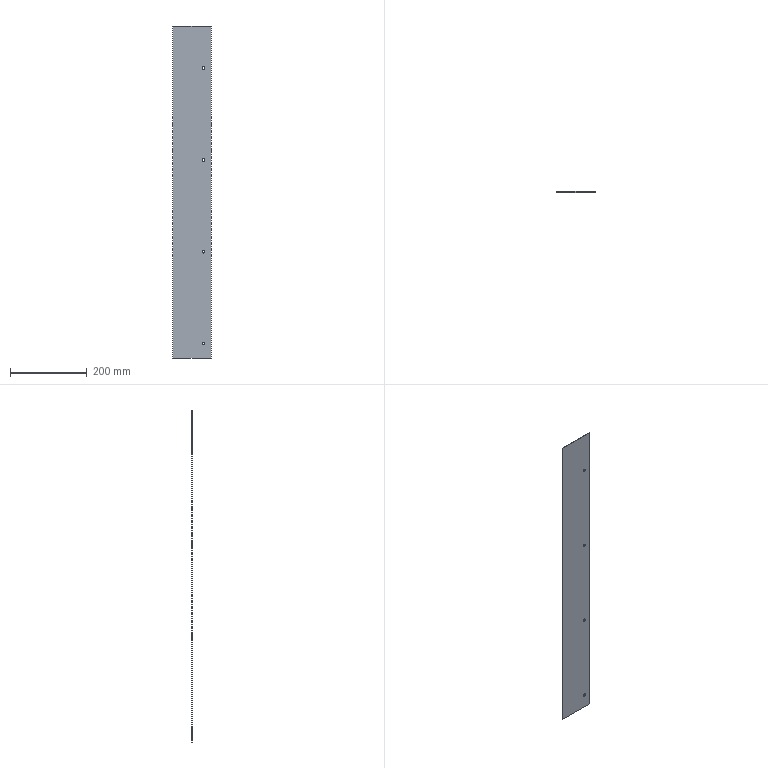Component | SolidWorks | 30-44A-1 | 1 solid | 14 faces | box 100 x 2 x 868 mm | volume 173292 mm3 | cylinder 8 | plane 6 | commonest cylinder face diameters 7 x8
STEP:
#1=COLOUR_RGB('',0.7922,0.8196,0.9333);
#2=FILL_AREA_STYLE_COLOUR('',#1);
#3=FILL_AREA_STYLE('',(#2));
#4=SURFACE_STYLE_FILL_AREA(#3);
#5=SURFACE_SIDE_STYLE('',(#4));
#6=SURFACE_STYLE_USAGE(.BOTH.,#5);
#7=PRESENTATION_STYLE_ASSIGNMENT((#6));
#8=CARTESIAN_POINT('',(10.731,28.038,-12.067));
#9=VERTEX_POINT('',#8);
#10=CARTESIAN_POINT('',(10.731,28.038,-12.343));
#11=VERTEX_POINT('',#10);
#12=CARTESIAN_POINT('',(10.731,28.038,-12.205));
#13=DIRECTION('',(-0.,-1.,0.));
#14=DIRECTION('',(0.,0.,-1.));
#15=AXIS2_PLACEMENT_3D('',#12,#13,#14);
#16=CIRCLE('',#15,0.1378);
#17=EDGE_CURVE('',#9,#11,#16,.T.);
#18=ORIENTED_EDGE('',*,*,#17,.T.);
#19=CARTESIAN_POINT('',(10.731,28.116,-12.343));
#20=VERTEX_POINT('',#19);
#21=CARTESIAN_POINT('',(10.731,27.723,-12.343));
#22=DIRECTION('',(0.,1.,-0.));
#23=VECTOR('',#22,39.37);
#24=LINE('',#21,#23);
#25=EDGE_CURVE('',#11,#20,#24,.T.);
#26=ORIENTED_EDGE('',*,*,#25,.T.);
#27=CARTESIAN_POINT('',(10.731,28.116,-12.067));
#28=VERTEX_POINT('',#27);
#29=CARTESIAN_POINT('',(10.731,28.116,-12.205));
#30=DIRECTION('',(0.,1.,-0.));
#31=DIRECTION('',(0.,0.,-1.));
#32=AXIS2_PLACEMENT_3D('',#29,#30,#31);
#33=CIRCLE('',#32,0.1378);
#34=EDGE_CURVE('',#20,#28,#33,.T.);
#35=ORIENTED_EDGE('',*,*,#34,.T.);
#36=CARTESIAN_POINT('',(10.731,27.723,-12.067));
#37=DIRECTION('',(0.,1.,-0.));
#38=VECTOR('',#37,39.37);
#39=LINE('',#36,#38);
#40=EDGE_CURVE('',#9,#28,#39,.T.);
#41=ORIENTED_EDGE('',*,*,#40,.F.);
#42=EDGE_LOOP('',(#18,#26,#35,#41));
#43=FACE_OUTER_BOUND('',#42,.T.);
#44=CARTESIAN_POINT('',(10.731,27.723,-12.205));
#45=DIRECTION('',(0.,1.,-0.));
#46=DIRECTION('',(0.,0.,1.));
#47=AXIS2_PLACEMENT_3D('',#44,#45,#46);
#48=CYLINDRICAL_SURFACE('',#47,0.1378);
#49=ADVANCED_FACE('',(#43),#48,.F.);
#50=CARTESIAN_POINT('',(10.731,28.038,-2.618));
#51=VERTEX_POINT('',#50);
#52=CARTESIAN_POINT('',(10.731,28.038,-2.894));
#53=VERTEX_POINT('',#52);
#54=CARTESIAN_POINT('',(10.731,28.038,-2.756));
#55=DIRECTION('',(-0.,-1.,0.));
#56=DIRECTION('',(0.,0.,-1.));
#57=AXIS2_PLACEMENT_3D('',#54,#55,#56);
#58=CIRCLE('',#57,0.1378);
#59=EDGE_CURVE('',#51,#53,#58,.T.);
#60=ORIENTED_EDGE('',*,*,#59,.T.);
#61=CARTESIAN_POINT('',(10.731,28.116,-2.894));
#62=VERTEX_POINT('',#61);
#63=CARTESIAN_POINT('',(10.731,27.723,-2.894));
#64=DIRECTION('',(0.,1.,-0.));
#65=VECTOR('',#64,39.37);
#66=LINE('',#63,#65);
#67=EDGE_CURVE('',#53,#62,#66,.T.);
#68=ORIENTED_EDGE('',*,*,#67,.T.);
#69=CARTESIAN_POINT('',(10.731,28.116,-2.618));
#70=VERTEX_POINT('',#69);
#71=CARTESIAN_POINT('',(10.731,28.116,-2.756));
#72=DIRECTION('',(0.,1.,-0.));
#73=DIRECTION('',(0.,0.,-1.));
#74=AXIS2_PLACEMENT_3D('',#71,#72,#73);
#75=CIRCLE('',#74,0.1378);
#76=EDGE_CURVE('',#62,#70,#75,.T.);
#77=ORIENTED_EDGE('',*,*,#76,.T.);
#78=CARTESIAN_POINT('',(10.731,27.723,-2.618));
#79=DIRECTION('',(0.,1.,-0.));
#80=VECTOR('',#79,39.37);
#81=LINE('',#78,#80);
#82=EDGE_CURVE('',#51,#70,#81,.T.);
#83=ORIENTED_EDGE('',*,*,#82,.F.);
#84=EDGE_LOOP('',(#60,#68,#77,#83));
#85=FACE_OUTER_BOUND('',#84,.T.);
#86=CARTESIAN_POINT('',(10.731,27.723,-2.756));
#87=DIRECTION('',(0.,1.,-0.));
#88=DIRECTION('',(0.,0.,1.));
#89=AXIS2_PLACEMENT_3D('',#86,#87,#88);
#90=CYLINDRICAL_SURFACE('',#89,0.1378);
#91=ADVANCED_FACE('',(#85),#90,.F.);
#92=CARTESIAN_POINT('',(10.731,28.038,-30.965));
#93=VERTEX_POINT('',#92);
#94=CARTESIAN_POINT('',(10.731,28.038,-31.24));
#95=VERTEX_POINT('',#94);
#96=CARTESIAN_POINT('',(10.731,28.038,-31.102));
#97=DIRECTION('',(-0.,-1.,0.));
#98=DIRECTION('',(0.,0.,-1.));
#99=AXIS2_PLACEMENT_3D('',#96,#97,#98);
#100=CIRCLE('',#99,0.1378);
#101=EDGE_CURVE('',#93,#95,#100,.T.);
#102=ORIENTED_EDGE('',*,*,#101,.T.);
#103=CARTESIAN_POINT('',(10.731,28.116,-31.24));
#104=VERTEX_POINT('',#103);
#105=CARTESIAN_POINT('',(10.731,27.723,-31.24));
#106=DIRECTION('',(0.,1.,-0.));
#107=VECTOR('',#106,39.37);
#108=LINE('',#105,#107);
#109=EDGE_CURVE('',#95,#104,#108,.T.);
#110=ORIENTED_EDGE('',*,*,#109,.T.);
#111=CARTESIAN_POINT('',(10.731,28.116,-30.965));
#112=VERTEX_POINT('',#111);
#113=CARTESIAN_POINT('',(10.731,28.116,-31.102));
#114=DIRECTION('',(0.,1.,-0.));
#115=DIRECTION('',(0.,0.,1.));
#116=AXIS2_PLACEMENT_3D('',#113,#114,#115);
#117=CIRCLE('',#116,0.1378);
#118=EDGE_CURVE('',#104,#112,#117,.T.);
#119=ORIENTED_EDGE('',*,*,#118,.T.);
#120=CARTESIAN_POINT('',(10.731,27.723,-30.965));
#121=DIRECTION('',(0.,1.,-0.));
#122=VECTOR('',#121,39.37);
#123=LINE('',#120,#122);
#124=EDGE_CURVE('',#93,#112,#123,.T.);
#125=ORIENTED_EDGE('',*,*,#124,.F.);
#126=EDGE_LOOP('',(#102,#110,#119,#125));
#127=FACE_OUTER_BOUND('',#126,.T.);
#128=CARTESIAN_POINT('',(10.731,27.723,-31.102));
#129=DIRECTION('',(0.,1.,-0.));
#130=DIRECTION('',(0.,0.,1.));
#131=AXIS2_PLACEMENT_3D('',#128,#129,#130);
#132=CYLINDRICAL_SURFACE('',#131,0.1378);
#133=ADVANCED_FACE('',(#127),#132,.F.);
#134=CARTESIAN_POINT('',(10.731,28.038,-21.516));
#135=VERTEX_POINT('',#134);
#136=CARTESIAN_POINT('',(10.731,28.038,-21.791));
#137=VERTEX_POINT('',#136);
#138=CARTESIAN_POINT('',(10.731,28.038,-21.654));
#139=DIRECTION('',(-0.,-1.,0.));
#140=DIRECTION('',(0.,0.,-1.));
#141=AXIS2_PLACEMENT_3D('',#138,#139,#140);
#142=CIRCLE('',#141,0.1378);
#143=EDGE_CURVE('',#135,#137,#142,.T.);
#144=ORIENTED_EDGE('',*,*,#143,.T.);
#145=CARTESIAN_POINT('',(10.731,28.116,-21.791));
#146=VERTEX_POINT('',#145);
#147=CARTESIAN_POINT('',(10.731,27.723,-21.791));
#148=DIRECTION('',(0.,1.,-0.));
#149=VECTOR('',#148,39.37);
#150=LINE('',#147,#149);
#151=EDGE_CURVE('',#137,#146,#150,.T.);
#152=ORIENTED_EDGE('',*,*,#151,.T.);
#153=CARTESIAN_POINT('',(10.731,28.116,-21.516));
#154=VERTEX_POINT('',#153);
#155=CARTESIAN_POINT('',(10.731,28.116,-21.654));
#156=DIRECTION('',(0.,1.,-0.));
#157=DIRECTION('',(0.,0.,1.));
#158=AXIS2_PLACEMENT_3D('',#155,#156,#157);
#159=CIRCLE('',#158,0.1378);
#160=EDGE_CURVE('',#146,#154,#159,.T.);
#161=ORIENTED_EDGE('',*,*,#160,.T.);
#162=CARTESIAN_POINT('',(10.731,27.723,-21.516));
#163=DIRECTION('',(0.,1.,-0.));
#164=VECTOR('',#163,39.37);
#165=LINE('',#162,#164);
#166=EDGE_CURVE('',#135,#154,#165,.T.);
#167=ORIENTED_EDGE('',*,*,#166,.F.);
#168=EDGE_LOOP('',(#144,#152,#161,#167));
#169=FACE_OUTER_BOUND('',#168,.T.);
#170=CARTESIAN_POINT('',(10.731,27.723,-21.654));
#171=DIRECTION('',(0.,1.,-0.));
#172=DIRECTION('',(0.,0.,1.));
#173=AXIS2_PLACEMENT_3D('',#170,#171,#172);
#174=CYLINDRICAL_SURFACE('',#173,0.1378);
#175=ADVANCED_FACE('',(#169),#174,.F.);
#176=CARTESIAN_POINT('',(11.519,28.116,1.575));
#177=VERTEX_POINT('',#176);
#178=CARTESIAN_POINT('',(7.582,28.116,1.575));
#179=VERTEX_POINT('',#178);
#180=CARTESIAN_POINT('',(11.519,28.116,1.575));
#181=DIRECTION('',(-1.,0.,-0.));
#182=VECTOR('',#181,39.37);
#183=LINE('',#180,#182);
#184=EDGE_CURVE('',#177,#179,#183,.T.);
#185=ORIENTED_EDGE('',*,*,#184,.T.);
#186=CARTESIAN_POINT('',(7.582,28.038,1.575));
#187=VERTEX_POINT('',#186);
#188=CARTESIAN_POINT('',(7.582,28.038,1.575));
#189=DIRECTION('',(0.,1.,-0.));
#190=VECTOR('',#189,39.37);
#191=LINE('',#188,#190);
#192=EDGE_CURVE('',#187,#179,#191,.T.);
#193=ORIENTED_EDGE('',*,*,#192,.F.);
#194=CARTESIAN_POINT('',(11.519,28.038,1.575));
#195=VERTEX_POINT('',#194);
#196=CARTESIAN_POINT('',(11.519,28.038,1.575));
#197=DIRECTION('',(-1.,0.,-0.));
#198=VECTOR('',#197,39.37);
#199=LINE('',#196,#198);
#200=EDGE_CURVE('',#195,#187,#199,.T.);
#201=ORIENTED_EDGE('',*,*,#200,.F.);
#202=CARTESIAN_POINT('',(11.519,28.038,1.575));
#203=DIRECTION('',(0.,1.,-0.));
#204=VECTOR('',#203,39.37);
#205=LINE('',#202,#204);
#206=EDGE_CURVE('',#195,#177,#205,.T.);
#207=ORIENTED_EDGE('',*,*,#206,.T.);
#208=EDGE_LOOP('',(#185,#193,#201,#207));
#209=FACE_OUTER_BOUND('',#208,.T.);
#210=CARTESIAN_POINT('',(11.519,28.038,1.575));
#211=DIRECTION('',(0.,-0.,-1.));
#212=DIRECTION('',(0.,1.,-0.));
#213=AXIS2_PLACEMENT_3D('',#210,#211,#212);
#214=PLANE('',#213);
#215=ADVANCED_FACE('',(#209),#214,.F.);
#216=CARTESIAN_POINT('',(7.582,28.116,-32.598));
#217=VERTEX_POINT('',#216);
#218=CARTESIAN_POINT('',(7.582,28.116,1.575));
#219=DIRECTION('',(0.,-0.,-1.));
#220=VECTOR('',#219,39.37);
#221=LINE('',#218,#220);
#222=EDGE_CURVE('',#179,#217,#221,.T.);
#223=ORIENTED_EDGE('',*,*,#222,.T.);
#224=CARTESIAN_POINT('',(7.582,28.038,-32.598));
#225=VERTEX_POINT('',#224);
#226=CARTESIAN_POINT('',(7.582,28.038,-32.598));
#227=DIRECTION('',(0.,1.,-0.));
#228=VECTOR('',#227,39.37);
#229=LINE('',#226,#228);
#230=EDGE_CURVE('',#225,#217,#229,.T.);
#231=ORIENTED_EDGE('',*,*,#230,.F.);
#232=CARTESIAN_POINT('',(7.582,28.038,1.575));
#233=DIRECTION('',(0.,-0.,-1.));
#234=VECTOR('',#233,39.37);
#235=LINE('',#232,#234);
#236=EDGE_CURVE('',#187,#225,#235,.T.);
#237=ORIENTED_EDGE('',*,*,#236,.F.);
#238=ORIENTED_EDGE('',*,*,#192,.T.);
#239=EDGE_LOOP('',(#223,#231,#237,#238));
#240=FACE_OUTER_BOUND('',#239,.T.);
#241=CARTESIAN_POINT('',(7.582,28.038,1.575));
#242=DIRECTION('',(1.,-0.,0.));
#243=DIRECTION('',(-0.,-1.,0.));
#244=AXIS2_PLACEMENT_3D('',#241,#242,#243);
#245=PLANE('',#244);
#246=ADVANCED_FACE('',(#240),#245,.F.);
#247=CARTESIAN_POINT('',(11.519,28.116,-32.598));
#248=VERTEX_POINT('',#247);
#249=CARTESIAN_POINT('',(11.519,28.116,-32.598));
#250=DIRECTION('',(1.,-0.,0.));
#251=VECTOR('',#250,39.37);
#252=LINE('',#249,#251);
#253=EDGE_CURVE('',#217,#248,#252,.T.);
#254=ORIENTED_EDGE('',*,*,#253,.T.);
#255=CARTESIAN_POINT('',(11.519,28.038,-32.598));
#256=VERTEX_POINT('',#255);
#257=CARTESIAN_POINT('',(11.519,28.038,-32.598));
#258=DIRECTION('',(0.,1.,-0.));
#259=VECTOR('',#258,39.37);
#260=LINE('',#257,#259);
#261=EDGE_CURVE('',#256,#248,#260,.T.);
#262=ORIENTED_EDGE('',*,*,#261,.F.);
#263=CARTESIAN_POINT('',(11.519,28.038,-32.598));
#264=DIRECTION('',(1.,-0.,0.));
#265=VECTOR('',#264,39.37);
#266=LINE('',#263,#265);
#267=EDGE_CURVE('',#225,#256,#266,.T.);
#268=ORIENTED_EDGE('',*,*,#267,.F.);
#269=ORIENTED_EDGE('',*,*,#230,.T.);
#270=EDGE_LOOP('',(#254,#262,#268,#269));
#271=FACE_OUTER_BOUND('',#270,.T.);
#272=CARTESIAN_POINT('',(11.519,28.038,-32.598));
#273=DIRECTION('',(0.,0.,1.));
#274=DIRECTION('',(-0.,-1.,0.));
#275=AXIS2_PLACEMENT_3D('',#272,#273,#274);
#276=PLANE('',#275);
#277=ADVANCED_FACE('',(#271),#276,.F.);
#278=CARTESIAN_POINT('',(11.519,28.116,1.575));
#279=DIRECTION('',(0.,0.,1.));
#280=VECTOR('',#279,39.37);
#281=LINE('',#278,#280);
#282=EDGE_CURVE('',#248,#177,#281,.T.);
#283=ORIENTED_EDGE('',*,*,#282,.T.);
#284=ORIENTED_EDGE('',*,*,#206,.F.);
#285=CARTESIAN_POINT('',(11.519,28.038,1.575));
#286=DIRECTION('',(0.,0.,1.));
#287=VECTOR('',#286,39.37);
#288=LINE('',#285,#287);
#289=EDGE_CURVE('',#256,#195,#288,.T.);
#290=ORIENTED_EDGE('',*,*,#289,.F.);
#291=ORIENTED_EDGE('',*,*,#261,.T.);
#292=EDGE_LOOP('',(#283,#284,#290,#291));
#293=FACE_OUTER_BOUND('',#292,.T.);
#294=CARTESIAN_POINT('',(11.519,28.038,1.575));
#295=DIRECTION('',(-1.,0.,-0.));
#296=DIRECTION('',(0.,1.,-0.));
#297=AXIS2_PLACEMENT_3D('',#294,#295,#296);
#298=PLANE('',#297);
#299=ADVANCED_FACE('',(#293),#298,.F.);
#300=ORIENTED_EDGE('',*,*,#17,.F.);
#301=CARTESIAN_POINT('',(10.731,28.038,-12.205));
#302=DIRECTION('',(-0.,-1.,0.));
#303=DIRECTION('',(0.,0.,-1.));
#304=AXIS2_PLACEMENT_3D('',#301,#302,#303);
#305=CIRCLE('',#304,0.1378);
#306=EDGE_CURVE('',#11,#9,#305,.T.);
#307=ORIENTED_EDGE('',*,*,#306,.F.);
#308=EDGE_LOOP('',(#300,#307));
#309=FACE_BOUND('',#308,.T.);
#310=ORIENTED_EDGE('',*,*,#59,.F.);
#311=CARTESIAN_POINT('',(10.731,28.038,-2.756));
#312=DIRECTION('',(-0.,-1.,0.));
#313=DIRECTION('',(0.,0.,-1.));
#314=AXIS2_PLACEMENT_3D('',#311,#312,#313);
#315=CIRCLE('',#314,0.1378);
#316=EDGE_CURVE('',#53,#51,#315,.T.);
#317=ORIENTED_EDGE('',*,*,#316,.F.);
#318=EDGE_LOOP('',(#310,#317));
#319=FACE_BOUND('',#318,.T.);
#320=ORIENTED_EDGE('',*,*,#101,.F.);
#321=CARTESIAN_POINT('',(10.731,28.038,-31.102));
#322=DIRECTION('',(-0.,-1.,0.));
#323=DIRECTION('',(0.,0.,-1.));
#324=AXIS2_PLACEMENT_3D('',#321,#322,#323);
#325=CIRCLE('',#324,0.1378);
#326=EDGE_CURVE('',#95,#93,#325,.T.);
#327=ORIENTED_EDGE('',*,*,#326,.F.);
#328=EDGE_LOOP('',(#320,#327));
#329=FACE_BOUND('',#328,.T.);
#330=ORIENTED_EDGE('',*,*,#143,.F.);
#331=CARTESIAN_POINT('',(10.731,28.038,-21.654));
#332=DIRECTION('',(-0.,-1.,0.));
#333=DIRECTION('',(0.,0.,-1.));
#334=AXIS2_PLACEMENT_3D('',#331,#332,#333);
#335=CIRCLE('',#334,0.1378);
#336=EDGE_CURVE('',#137,#135,#335,.T.);
#337=ORIENTED_EDGE('',*,*,#336,.F.);
#338=EDGE_LOOP('',(#330,#337));
#339=FACE_BOUND('',#338,.T.);
#340=ORIENTED_EDGE('',*,*,#200,.T.);
#341=ORIENTED_EDGE('',*,*,#236,.T.);
#342=ORIENTED_EDGE('',*,*,#267,.T.);
#343=ORIENTED_EDGE('',*,*,#289,.T.);
#344=EDGE_LOOP('',(#340,#341,#342,#343));
#345=FACE_OUTER_BOUND('',#344,.T.);
#346=CARTESIAN_POINT('',(7.582,28.038,1.575));
#347=DIRECTION('',(-0.,-1.,0.));
#348=DIRECTION('',(0.,-0.,-1.));
#349=AXIS2_PLACEMENT_3D('',#346,#347,#348);
#350=PLANE('',#349);
#351=ADVANCED_FACE('',(#309,#319,#329,#339,#345),#350,.T.);
#352=CARTESIAN_POINT('',(10.731,28.116,-12.205));
#353=DIRECTION('',(0.,1.,-0.));
#354=DIRECTION('',(0.,0.,-1.));
#355=AXIS2_PLACEMENT_3D('',#352,#353,#354);
#356=CIRCLE('',#355,0.1378);
#357=EDGE_CURVE('',#28,#20,#356,.T.);
#358=ORIENTED_EDGE('',*,*,#357,.F.);
#359=ORIENTED_EDGE('',*,*,#34,.F.);
#360=EDGE_LOOP('',(#358,#359));
#361=FACE_BOUND('',#360,.T.);
#362=CARTESIAN_POINT('',(10.731,28.116,-2.756));
#363=DIRECTION('',(0.,1.,-0.));
#364=DIRECTION('',(0.,0.,-1.));
#365=AXIS2_PLACEMENT_3D('',#362,#363,#364);
#366=CIRCLE('',#365,0.1378);
#367=EDGE_CURVE('',#70,#62,#366,.T.);
#368=ORIENTED_EDGE('',*,*,#367,.F.);
#369=ORIENTED_EDGE('',*,*,#76,.F.);
#370=EDGE_LOOP('',(#368,#369));
#371=FACE_BOUND('',#370,.T.);
#372=CARTESIAN_POINT('',(10.731,28.116,-31.102));
#373=DIRECTION('',(0.,1.,-0.));
#374=DIRECTION('',(0.,0.,1.));
#375=AXIS2_PLACEMENT_3D('',#372,#373,#374);
#376=CIRCLE('',#375,0.1378);
#377=EDGE_CURVE('',#112,#104,#376,.T.);
#378=ORIENTED_EDGE('',*,*,#377,.F.);
#379=ORIENTED_EDGE('',*,*,#118,.F.);
#380=EDGE_LOOP('',(#378,#379));
#381=FACE_BOUND('',#380,.T.);
#382=CARTESIAN_POINT('',(10.731,28.116,-21.654));
#383=DIRECTION('',(0.,1.,-0.));
#384=DIRECTION('',(0.,0.,1.));
#385=AXIS2_PLACEMENT_3D('',#382,#383,#384);
#386=CIRCLE('',#385,0.1378);
#387=EDGE_CURVE('',#154,#146,#386,.T.);
#388=ORIENTED_EDGE('',*,*,#387,.F.);
#389=ORIENTED_EDGE('',*,*,#160,.F.);
#390=EDGE_LOOP('',(#388,#389));
#391=FACE_BOUND('',#390,.T.);
#392=ORIENTED_EDGE('',*,*,#184,.F.);
#393=ORIENTED_EDGE('',*,*,#282,.F.);
#394=ORIENTED_EDGE('',*,*,#253,.F.);
#395=ORIENTED_EDGE('',*,*,#222,.F.);
#396=EDGE_LOOP('',(#392,#393,#394,#395));
#397=FACE_OUTER_BOUND('',#396,.T.);
#398=CARTESIAN_POINT('',(7.582,28.116,1.575));
#399=DIRECTION('',(-0.,-1.,0.));
#400=DIRECTION('',(0.,-0.,-1.));
#401=AXIS2_PLACEMENT_3D('',#398,#399,#400);
#402=PLANE('',#401);
#403=ADVANCED_FACE('',(#361,#371,#381,#391,#397),#402,.F.);
#404=ORIENTED_EDGE('',*,*,#151,.F.);
#405=ORIENTED_EDGE('',*,*,#336,.T.);
#406=ORIENTED_EDGE('',*,*,#166,.T.);
#407=ORIENTED_EDGE('',*,*,#387,.T.);
#408=EDGE_LOOP('',(#404,#405,#406,#407));
#409=FACE_OUTER_BOUND('',#408,.T.);
#410=CARTESIAN_POINT('',(10.731,27.723,-21.654));
#411=DIRECTION('',(0.,1.,-0.));
#412=DIRECTION('',(0.,0.,1.));
#413=AXIS2_PLACEMENT_3D('',#410,#411,#412);
#414=CYLINDRICAL_SURFACE('',#413,0.1378);
#415=ADVANCED_FACE('',(#409),#414,.F.);
#416=ORIENTED_EDGE('',*,*,#109,.F.);
#417=ORIENTED_EDGE('',*,*,#326,.T.);
#418=ORIENTED_EDGE('',*,*,#124,.T.);
#419=ORIENTED_EDGE('',*,*,#377,.T.);
#420=EDGE_LOOP('',(#416,#417,#418,#419));
#421=FACE_OUTER_BOUND('',#420,.T.);
#422=CARTESIAN_POINT('',(10.731,27.723,-31.102));
#423=DIRECTION('',(0.,1.,-0.));
#424=DIRECTION('',(0.,0.,1.));
#425=AXIS2_PLACEMENT_3D('',#422,#423,#424);
#426=CYLINDRICAL_SURFACE('',#425,0.1378);
#427=ADVANCED_FACE('',(#421),#426,.F.);
#428=ORIENTED_EDGE('',*,*,#67,.F.);
#429=ORIENTED_EDGE('',*,*,#316,.T.);
#430=ORIENTED_EDGE('',*,*,#82,.T.);
#431=ORIENTED_EDGE('',*,*,#367,.T.);
#432=EDGE_LOOP('',(#428,#429,#430,#431));
#433=FACE_OUTER_BOUND('',#432,.T.);
#434=CARTESIAN_POINT('',(10.731,27.723,-2.756));
#435=DIRECTION('',(0.,1.,-0.));
#436=DIRECTION('',(0.,0.,1.));
#437=AXIS2_PLACEMENT_3D('',#434,#435,#436);
#438=CYLINDRICAL_SURFACE('',#437,0.1378);
#439=ADVANCED_FACE('',(#433),#438,.F.);
#440=ORIENTED_EDGE('',*,*,#25,.F.);
#441=ORIENTED_EDGE('',*,*,#306,.T.);
#442=ORIENTED_EDGE('',*,*,#40,.T.);
#443=ORIENTED_EDGE('',*,*,#357,.T.);
#444=EDGE_LOOP('',(#440,#441,#442,#443));
#445=FACE_OUTER_BOUND('',#444,.T.);
#446=CARTESIAN_POINT('',(10.731,27.723,-12.205));
#447=DIRECTION('',(0.,1.,-0.));
#448=DIRECTION('',(0.,0.,1.));
#449=AXIS2_PLACEMENT_3D('',#446,#447,#448);
#450=CYLINDRICAL_SURFACE('',#449,0.1378);
#451=ADVANCED_FACE('',(#445),#450,.F.);
#452=CLOSED_SHELL('',(#49,#91,#133,#175,#215,#246,#277,#299,#351,#403,#415,#427,#439,#451));
#453=MANIFOLD_SOLID_BREP('',#452);
#454=STYLED_ITEM('',(#7),#453);
#455=(LENGTH_UNIT()NAMED_UNIT(*)SI_UNIT($,.METRE.));
#456=LENGTH_MEASURE_WITH_UNIT(LENGTH_MEASURE(0.0254),#455);
#457=DIMENSIONAL_EXPONENTS(1.,0.,0.,0.,0.,0.,0.);
#458=(CONVERSION_BASED_UNIT('',#456)LENGTH_UNIT()NAMED_UNIT(#457));
#459=UNCERTAINTY_MEASURE_WITH_UNIT(LENGTH_MEASURE(0.00001),#458,'','');
#460=(NAMED_UNIT(*)PLANE_ANGLE_UNIT()SI_UNIT($,.RADIAN.));
#461=(NAMED_UNIT(*)SI_UNIT($,.STERADIAN.)SOLID_ANGLE_UNIT());
#462=(GEOMETRIC_REPRESENTATION_CONTEXT(3)GLOBAL_UNCERTAINTY_ASSIGNED_CONTEXT((#459))GLOBAL_UNIT_ASSIGNED_CONTEXT((#458,#460,#461))REPRESENTATION_CONTEXT('',''));
#463=MECHANICAL_DESIGN_GEOMETRIC_PRESENTATION_REPRESENTATION('',(#454),#462);
#464=CARTESIAN_POINT('',(0.,0.,0.));
#465=DIRECTION('',(0.,0.,1.));
#466=DIRECTION('',(1.,0.,0.));
#467=AXIS2_PLACEMENT_3D('',#464,#465,#466);
#468=(LENGTH_UNIT()NAMED_UNIT(*)SI_UNIT($,.METRE.));
#469=LENGTH_MEASURE_WITH_UNIT(LENGTH_MEASURE(0.0254),#468);
#470=DIMENSIONAL_EXPONENTS(1.,0.,0.,0.,0.,0.,0.);
#471=(CONVERSION_BASED_UNIT('',#469)LENGTH_UNIT()NAMED_UNIT(#470));
#472=UNCERTAINTY_MEASURE_WITH_UNIT(LENGTH_MEASURE(0.00001),#471,'','');
#473=(NAMED_UNIT(*)PLANE_ANGLE_UNIT()SI_UNIT($,.RADIAN.));
#474=(NAMED_UNIT(*)SI_UNIT($,.STERADIAN.)SOLID_ANGLE_UNIT());
#475=(GEOMETRIC_REPRESENTATION_CONTEXT(3)GLOBAL_UNCERTAINTY_ASSIGNED_CONTEXT((#472))GLOBAL_UNIT_ASSIGNED_CONTEXT((#471,#473,#474))REPRESENTATION_CONTEXT('',''));
#476=ADVANCED_BREP_SHAPE_REPRESENTATION('',(#453,#467),#475);
#477=PRESENTATION_LAYER_ASSIGNMENT('','',(#454));